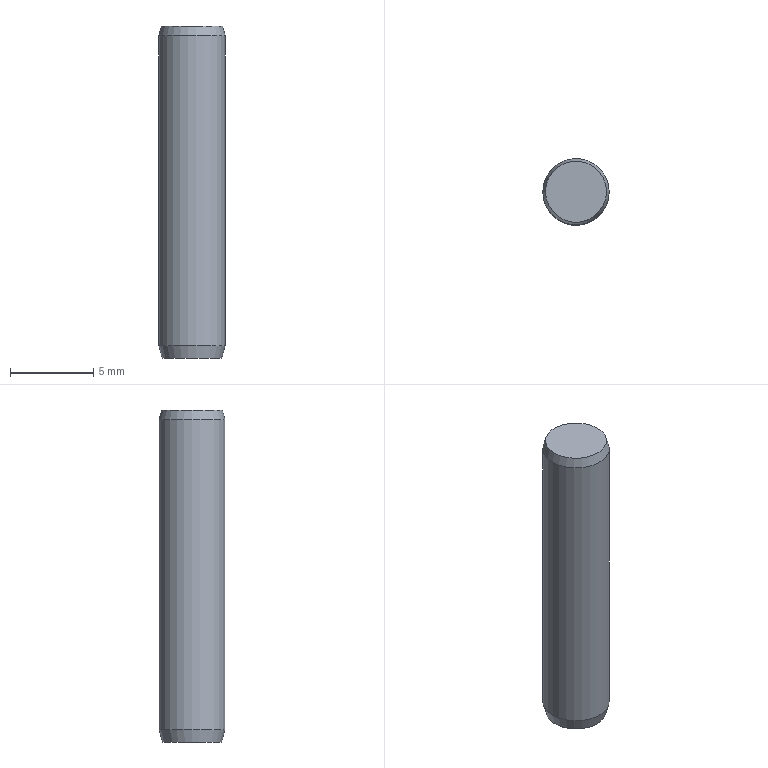Component | NX | CYL_PIN_2 | 1 solid | 5 faces | box 4 x 4 x 20 mm | volume 250 mm3 | plane 2 | cone 2 | cylinder 1 | commonest cylinder face diameters 4 x1
STEP:
#1=CARTESIAN_POINT('',(0.,0.,0.));
#2=DIRECTION('',(0.,0.,1.));
#3=DIRECTION('',(1.,0.,0.));
#4=AXIS2_PLACEMENT_3D('',#1,#2,#3);
#5=CARTESIAN_POINT('',(31.835,126.391,92.));
#6=VERTEX_POINT('',#5);
#7=CARTESIAN_POINT('',(29.996,126.391,92.));
#8=DIRECTION('',(0.,0.,1.));
#9=DIRECTION('',(1.,-0.0001511,0.));
#10=AXIS2_PLACEMENT_3D('',#7,#8,#9);
#11=CIRCLE('',#10,1.839);
#12=CARTESIAN_POINT('',(29.996,128.391,92.));
#13=DIRECTION('',(0.,0.,1.));
#14=DIRECTION('',(1.,-0.0001511,0.));
#15=AXIS2_PLACEMENT_3D('',#12,#13,#14);
#16=PLANE('',#15);
#17=CARTESIAN_POINT('',(0.,-2.));
#18=DIRECTION('',(1.,-0.));
#19=AXIS2_PLACEMENT_2D('',#17,#18);
#20=CIRCLE('',#19,1.839);
#21=(GEOMETRIC_REPRESENTATION_CONTEXT(2)PARAMETRIC_REPRESENTATION_CONTEXT()REPRESENTATION_CONTEXT('',''));
#22=DEFINITIONAL_REPRESENTATION('',(#20),#21);
#23=PCURVE('',#16,#22);
#24=CARTESIAN_POINT('',(29.996,126.391,91.4));
#25=DIRECTION('',(0.,0.,-1.));
#26=DIRECTION('',(-1.,0.0001511,0.));
#27=AXIS2_PLACEMENT_3D('',#24,#25,#26);
#28=CONICAL_SURFACE('',#27,2.,0.2618);
#29=CARTESIAN_POINT('',(9.425,-0.6));
#30=DIRECTION('',(-1.,0.));
#31=VECTOR('',#30,1.);
#32=LINE('',#29,#31);
#33=(GEOMETRIC_REPRESENTATION_CONTEXT(2)PARAMETRIC_REPRESENTATION_CONTEXT()REPRESENTATION_CONTEXT('',''));
#34=DEFINITIONAL_REPRESENTATION('',(#32),#33);
#35=PCURVE('',#28,#34);
#36=SURFACE_CURVE('',#11,(#23,#35),.PCURVE_S1.);
#37=EDGE_CURVE('',#6,#6,#36,.T.);
#38=ORIENTED_EDGE('',*,*,#37,.T.);
#39=EDGE_LOOP('',(#38));
#40=FACE_BOUND('',#39,.T.);
#41=ADVANCED_FACE('',(#40),#16,.T.);
#42=CARTESIAN_POINT('',(28.196,126.392,72.));
#43=VERTEX_POINT('',#42);
#44=CARTESIAN_POINT('',(29.996,126.391,72.));
#45=DIRECTION('',(0.,0.,-1.));
#46=DIRECTION('',(-1.,0.0001511,0.));
#47=AXIS2_PLACEMENT_3D('',#44,#45,#46);
#48=CIRCLE('',#47,1.8);
#49=CARTESIAN_POINT('',(29.996,126.391,72.));
#50=DIRECTION('',(0.,0.,-1.));
#51=DIRECTION('',(-1.,0.0001511,0.));
#52=AXIS2_PLACEMENT_3D('',#49,#50,#51);
#53=PLANE('',#52);
#54=CARTESIAN_POINT('',(0.,0.));
#55=DIRECTION('',(1.,0.));
#56=AXIS2_PLACEMENT_2D('',#54,#55);
#57=CIRCLE('',#56,1.8);
#58=(GEOMETRIC_REPRESENTATION_CONTEXT(2)PARAMETRIC_REPRESENTATION_CONTEXT()REPRESENTATION_CONTEXT('',''));
#59=DEFINITIONAL_REPRESENTATION('',(#57),#58);
#60=PCURVE('',#53,#59);
#61=CARTESIAN_POINT('',(29.996,126.391,72.));
#62=DIRECTION('',(0.,0.,1.));
#63=DIRECTION('',(1.,-0.0001511,0.));
#64=AXIS2_PLACEMENT_3D('',#61,#62,#63);
#65=CONICAL_SURFACE('',#64,1.8,0.2618);
#66=CARTESIAN_POINT('',(9.425,0.));
#67=DIRECTION('',(-1.,0.));
#68=VECTOR('',#67,1.);
#69=LINE('',#66,#68);
#70=(GEOMETRIC_REPRESENTATION_CONTEXT(2)PARAMETRIC_REPRESENTATION_CONTEXT()REPRESENTATION_CONTEXT('',''));
#71=DEFINITIONAL_REPRESENTATION('',(#69),#70);
#72=PCURVE('',#65,#71);
#73=SURFACE_CURVE('',#48,(#60,#72),.PCURVE_S1.);
#74=EDGE_CURVE('',#43,#43,#73,.T.);
#75=ORIENTED_EDGE('',*,*,#74,.T.);
#76=EDGE_LOOP('',(#75));
#77=FACE_BOUND('',#76,.T.);
#78=ADVANCED_FACE('',(#77),#53,.T.);
#79=CARTESIAN_POINT('',(27.996,126.392,72.746));
#80=VERTEX_POINT('',#79);
#81=CARTESIAN_POINT('',(29.996,126.391,72.746));
#82=DIRECTION('',(0.,0.,1.));
#83=DIRECTION('',(-1.,0.0001511,0.));
#84=AXIS2_PLACEMENT_3D('',#81,#82,#83);
#85=CIRCLE('',#84,2.);
#86=CARTESIAN_POINT('',(29.996,126.391,72.));
#87=DIRECTION('',(0.,0.,-1.));
#88=DIRECTION('',(-1.,0.0001511,0.));
#89=AXIS2_PLACEMENT_3D('',#86,#87,#88);
#90=CYLINDRICAL_SURFACE('',#89,2.);
#91=CARTESIAN_POINT('',(6.283,-0.7464));
#92=DIRECTION('',(-1.,0.));
#93=VECTOR('',#92,1.);
#94=LINE('',#91,#93);
#95=(GEOMETRIC_REPRESENTATION_CONTEXT(2)PARAMETRIC_REPRESENTATION_CONTEXT()REPRESENTATION_CONTEXT('',''));
#96=DEFINITIONAL_REPRESENTATION('',(#94),#95);
#97=PCURVE('',#90,#96);
#98=CARTESIAN_POINT('',(3.142,0.7464));
#99=DIRECTION('',(1.,0.));
#100=VECTOR('',#99,1.);
#101=LINE('',#98,#100);
#102=(GEOMETRIC_REPRESENTATION_CONTEXT(2)PARAMETRIC_REPRESENTATION_CONTEXT()REPRESENTATION_CONTEXT('',''));
#103=DEFINITIONAL_REPRESENTATION('',(#101),#102);
#104=PCURVE('',#65,#103);
#105=SURFACE_CURVE('',#85,(#97,#104),.PCURVE_S1.);
#106=EDGE_CURVE('',#80,#80,#105,.T.);
#107=ORIENTED_EDGE('',*,*,#106,.T.);
#108=CARTESIAN_POINT('',(27.996,126.392,91.4));
#109=VERTEX_POINT('',#108);
#110=CARTESIAN_POINT('',(27.996,126.392,91.4));
#111=CARTESIAN_POINT('',(27.996,126.392,72.746));
#112=B_SPLINE_CURVE_WITH_KNOTS('',1,(#110,#111),.UNSPECIFIED.,.F.,.F.,(2,2),(-19.4,-0.7464),.PIECEWISE_BEZIER_KNOTS.);
#113=CARTESIAN_POINT('',(0.,0.));
#114=DIRECTION('',(0.,1.));
#115=VECTOR('',#114,1.);
#116=LINE('',#113,#115);
#117=(GEOMETRIC_REPRESENTATION_CONTEXT(2)PARAMETRIC_REPRESENTATION_CONTEXT()REPRESENTATION_CONTEXT('',''));
#118=DEFINITIONAL_REPRESENTATION('',(#116),#117);
#119=PCURVE('',#90,#118);
#120=CARTESIAN_POINT('',(6.283,0.));
#121=DIRECTION('',(0.,1.));
#122=VECTOR('',#121,1.);
#123=LINE('',#120,#122);
#124=(GEOMETRIC_REPRESENTATION_CONTEXT(2)PARAMETRIC_REPRESENTATION_CONTEXT()REPRESENTATION_CONTEXT('',''));
#125=DEFINITIONAL_REPRESENTATION('',(#123),#124);
#126=PCURVE('',#90,#125);
#127=SEAM_CURVE('',#112,(#119,#126),.PCURVE_S1.);
#128=EDGE_CURVE('',#109,#80,#127,.T.);
#129=ORIENTED_EDGE('',*,*,#128,.F.);
#130=CARTESIAN_POINT('',(31.996,126.391,91.4));
#131=VERTEX_POINT('',#130);
#132=CARTESIAN_POINT('',(29.996,126.391,91.4));
#133=DIRECTION('',(0.,0.,-1.));
#134=DIRECTION('',(1.,-0.0001511,0.));
#135=AXIS2_PLACEMENT_3D('',#132,#133,#134);
#136=CIRCLE('',#135,2.);
#137=CARTESIAN_POINT('',(-3.142,-19.4));
#138=DIRECTION('',(1.,0.));
#139=VECTOR('',#138,1.);
#140=LINE('',#137,#139);
#141=(GEOMETRIC_REPRESENTATION_CONTEXT(2)PARAMETRIC_REPRESENTATION_CONTEXT()REPRESENTATION_CONTEXT('',''));
#142=DEFINITIONAL_REPRESENTATION('',(#140),#141);
#143=PCURVE('',#90,#142);
#144=CARTESIAN_POINT('',(3.142,0.));
#145=DIRECTION('',(1.,0.));
#146=VECTOR('',#145,1.);
#147=LINE('',#144,#146);
#148=(GEOMETRIC_REPRESENTATION_CONTEXT(2)PARAMETRIC_REPRESENTATION_CONTEXT()REPRESENTATION_CONTEXT('',''));
#149=DEFINITIONAL_REPRESENTATION('',(#147),#148);
#150=PCURVE('',#28,#149);
#151=SURFACE_CURVE('',#136,(#143,#150),.PCURVE_S1.);
#152=EDGE_CURVE('',#109,#131,#151,.T.);
#153=ORIENTED_EDGE('',*,*,#152,.T.);
#154=CARTESIAN_POINT('',(29.996,126.391,91.4));
#155=DIRECTION('',(0.,0.,-1.));
#156=DIRECTION('',(1.,-0.0001511,0.));
#157=AXIS2_PLACEMENT_3D('',#154,#155,#156);
#158=CIRCLE('',#157,2.);
#159=CARTESIAN_POINT('',(3.142,-19.4));
#160=DIRECTION('',(1.,0.));
#161=VECTOR('',#160,1.);
#162=LINE('',#159,#161);
#163=(GEOMETRIC_REPRESENTATION_CONTEXT(2)PARAMETRIC_REPRESENTATION_CONTEXT()REPRESENTATION_CONTEXT('',''));
#164=DEFINITIONAL_REPRESENTATION('',(#162),#163);
#165=PCURVE('',#90,#164);
#166=CARTESIAN_POINT('',(3.142,0.));
#167=DIRECTION('',(1.,0.));
#168=VECTOR('',#167,1.);
#169=LINE('',#166,#168);
#170=(GEOMETRIC_REPRESENTATION_CONTEXT(2)PARAMETRIC_REPRESENTATION_CONTEXT()REPRESENTATION_CONTEXT('',''));
#171=DEFINITIONAL_REPRESENTATION('',(#169),#170);
#172=PCURVE('',#28,#171);
#173=SURFACE_CURVE('',#158,(#165,#172),.PCURVE_S1.);
#174=EDGE_CURVE('',#131,#109,#173,.T.);
#175=ORIENTED_EDGE('',*,*,#174,.T.);
#176=ORIENTED_EDGE('',*,*,#128,.T.);
#177=EDGE_LOOP('',(#107,#129,#153,#175,#176));
#178=FACE_BOUND('',#177,.T.);
#179=ADVANCED_FACE('',(#178),#90,.T.);
#180=ORIENTED_EDGE('',*,*,#37,.F.);
#181=CARTESIAN_POINT('',(31.835,126.391,92.));
#182=CARTESIAN_POINT('',(31.996,126.391,91.4));
#183=B_SPLINE_CURVE_WITH_KNOTS('',1,(#181,#182),.UNSPECIFIED.,.F.,.F.,(2,2),(-0.6212,0.),.PIECEWISE_BEZIER_KNOTS.);
#184=CARTESIAN_POINT('',(9.425,0.));
#185=DIRECTION('',(0.,1.));
#186=VECTOR('',#185,1.);
#187=LINE('',#184,#186);
#188=(GEOMETRIC_REPRESENTATION_CONTEXT(2)PARAMETRIC_REPRESENTATION_CONTEXT()REPRESENTATION_CONTEXT('',''));
#189=DEFINITIONAL_REPRESENTATION('',(#187),#188);
#190=PCURVE('',#28,#189);
#191=CARTESIAN_POINT('',(3.142,0.));
#192=DIRECTION('',(0.,1.));
#193=VECTOR('',#192,1.);
#194=LINE('',#191,#193);
#195=(GEOMETRIC_REPRESENTATION_CONTEXT(2)PARAMETRIC_REPRESENTATION_CONTEXT()REPRESENTATION_CONTEXT('',''));
#196=DEFINITIONAL_REPRESENTATION('',(#194),#195);
#197=PCURVE('',#28,#196);
#198=SEAM_CURVE('',#183,(#190,#197),.PCURVE_S1.);
#199=EDGE_CURVE('',#6,#131,#198,.T.);
#200=ORIENTED_EDGE('',*,*,#199,.T.);
#201=ORIENTED_EDGE('',*,*,#152,.F.);
#202=ORIENTED_EDGE('',*,*,#174,.F.);
#203=ORIENTED_EDGE('',*,*,#199,.F.);
#204=EDGE_LOOP('',(#180,#200,#201,#202,#203));
#205=FACE_BOUND('',#204,.T.);
#206=ADVANCED_FACE('',(#205),#28,.T.);
#207=ORIENTED_EDGE('',*,*,#106,.F.);
#208=CARTESIAN_POINT('',(28.196,126.392,72.));
#209=CARTESIAN_POINT('',(27.996,126.392,72.746));
#210=B_SPLINE_CURVE_WITH_KNOTS('',1,(#208,#209),.UNSPECIFIED.,.F.,.F.,(2,2),(0.,0.7727),.PIECEWISE_BEZIER_KNOTS.);
#211=CARTESIAN_POINT('',(3.142,0.));
#212=DIRECTION('',(0.,1.));
#213=VECTOR('',#212,1.);
#214=LINE('',#211,#213);
#215=(GEOMETRIC_REPRESENTATION_CONTEXT(2)PARAMETRIC_REPRESENTATION_CONTEXT()REPRESENTATION_CONTEXT('',''));
#216=DEFINITIONAL_REPRESENTATION('',(#214),#215);
#217=PCURVE('',#65,#216);
#218=CARTESIAN_POINT('',(9.425,0.));
#219=DIRECTION('',(0.,1.));
#220=VECTOR('',#219,1.);
#221=LINE('',#218,#220);
#222=(GEOMETRIC_REPRESENTATION_CONTEXT(2)PARAMETRIC_REPRESENTATION_CONTEXT()REPRESENTATION_CONTEXT('',''));
#223=DEFINITIONAL_REPRESENTATION('',(#221),#222);
#224=PCURVE('',#65,#223);
#225=SEAM_CURVE('',#210,(#217,#224),.PCURVE_S1.);
#226=EDGE_CURVE('',#43,#80,#225,.T.);
#227=ORIENTED_EDGE('',*,*,#226,.F.);
#228=ORIENTED_EDGE('',*,*,#74,.F.);
#229=ORIENTED_EDGE('',*,*,#226,.T.);
#230=EDGE_LOOP('',(#207,#227,#228,#229));
#231=FACE_BOUND('',#230,.T.);
#232=ADVANCED_FACE('',(#231),#65,.T.);
#233=CLOSED_SHELL('',(#41,#78,#179,#206,#232));
#234=MANIFOLD_SOLID_BREP('',#233);
#235=(LENGTH_UNIT()NAMED_UNIT(*)SI_UNIT(.MILLI.,.METRE.));
#236=UNCERTAINTY_MEASURE_WITH_UNIT(LENGTH_MEASURE(0.00001),#235,'','');
#237=(NAMED_UNIT(*)PLANE_ANGLE_UNIT()SI_UNIT($,.RADIAN.));
#238=(NAMED_UNIT(*)SI_UNIT($,.STERADIAN.)SOLID_ANGLE_UNIT());
#239=(GEOMETRIC_REPRESENTATION_CONTEXT(3)GLOBAL_UNCERTAINTY_ASSIGNED_CONTEXT((#236))GLOBAL_UNIT_ASSIGNED_CONTEXT((#235,#237,#238))REPRESENTATION_CONTEXT('',''));
#240=ADVANCED_BREP_SHAPE_REPRESENTATION('',(#4,#234),#239);